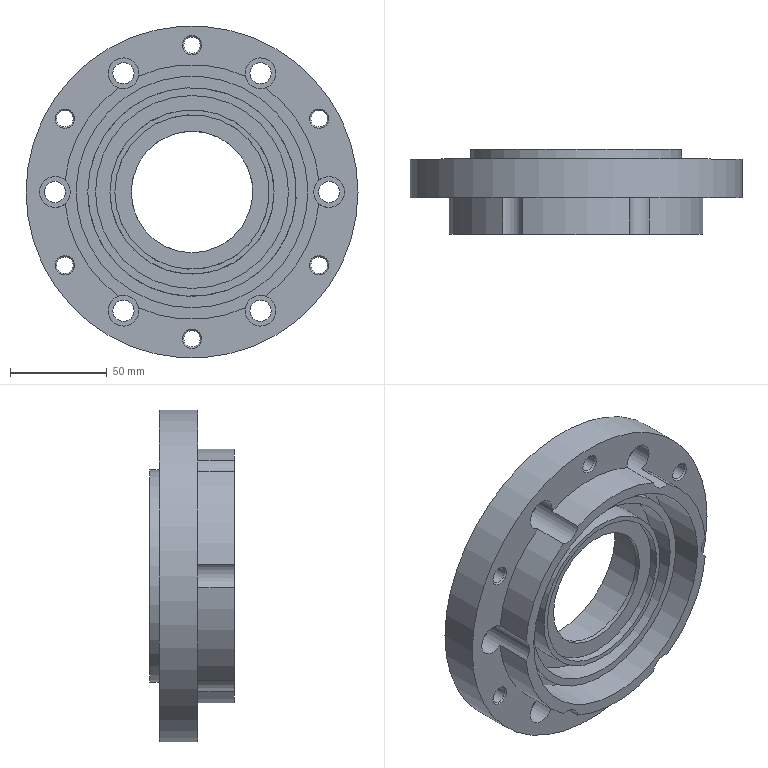Component | NX | LOWER_END_CAP | 1 solid | 63 faces | volume 395009 mm3 | cylinder 34 | plane 17 | cone 12 | commonest cylinder face diameters 132 x6 11 x6 16 x6 8.5 x6 80 x2 108 x1 63 x1 172 x1